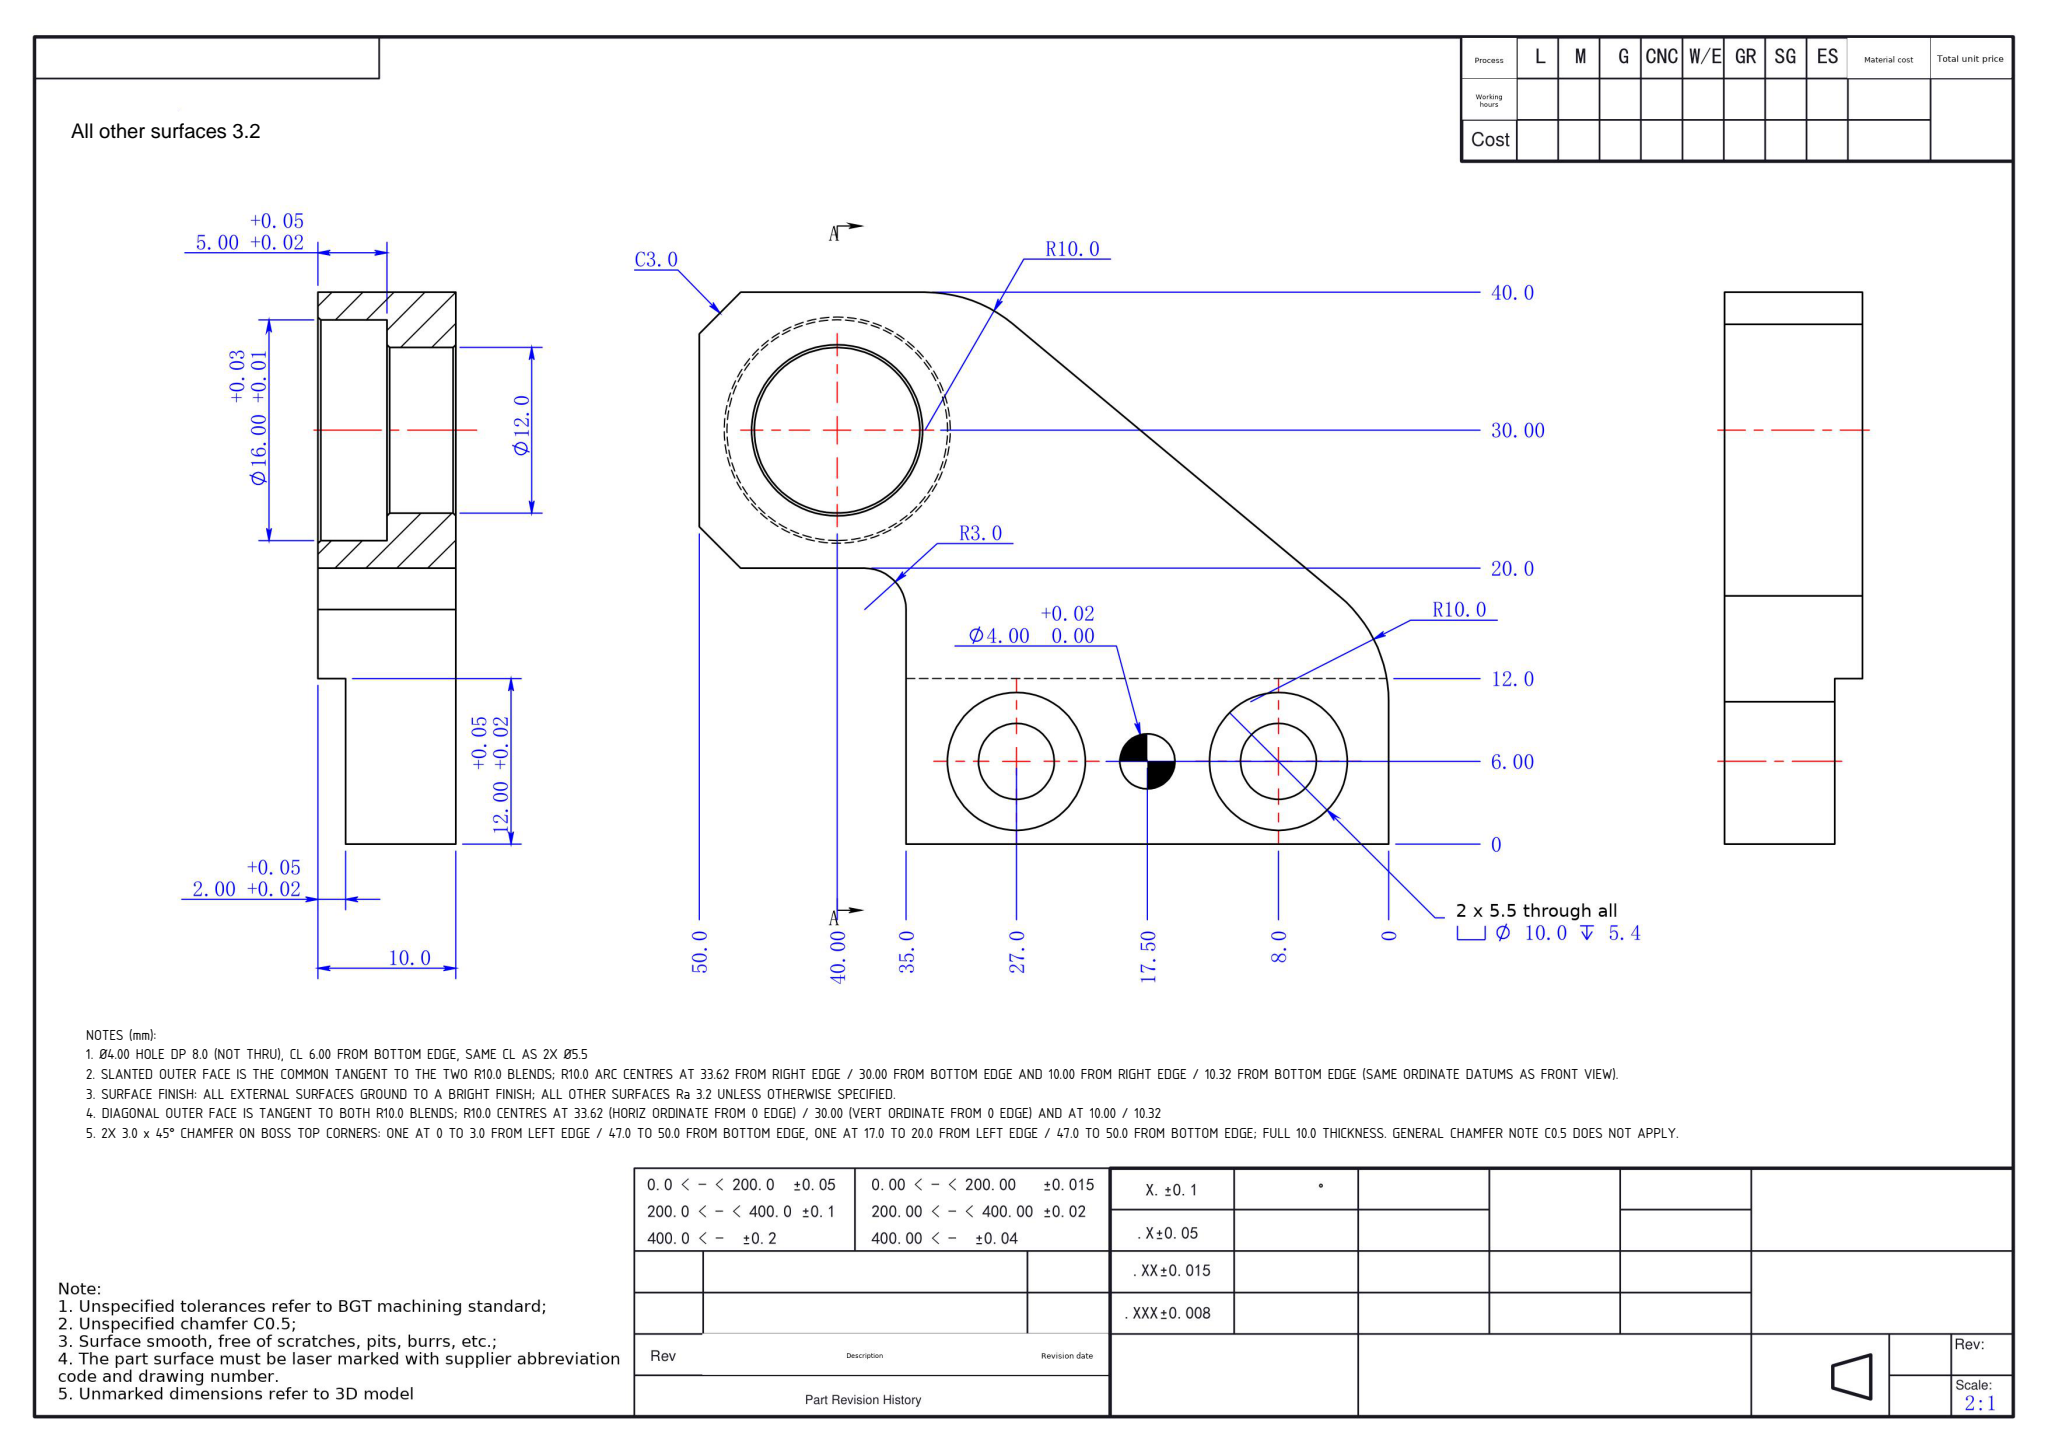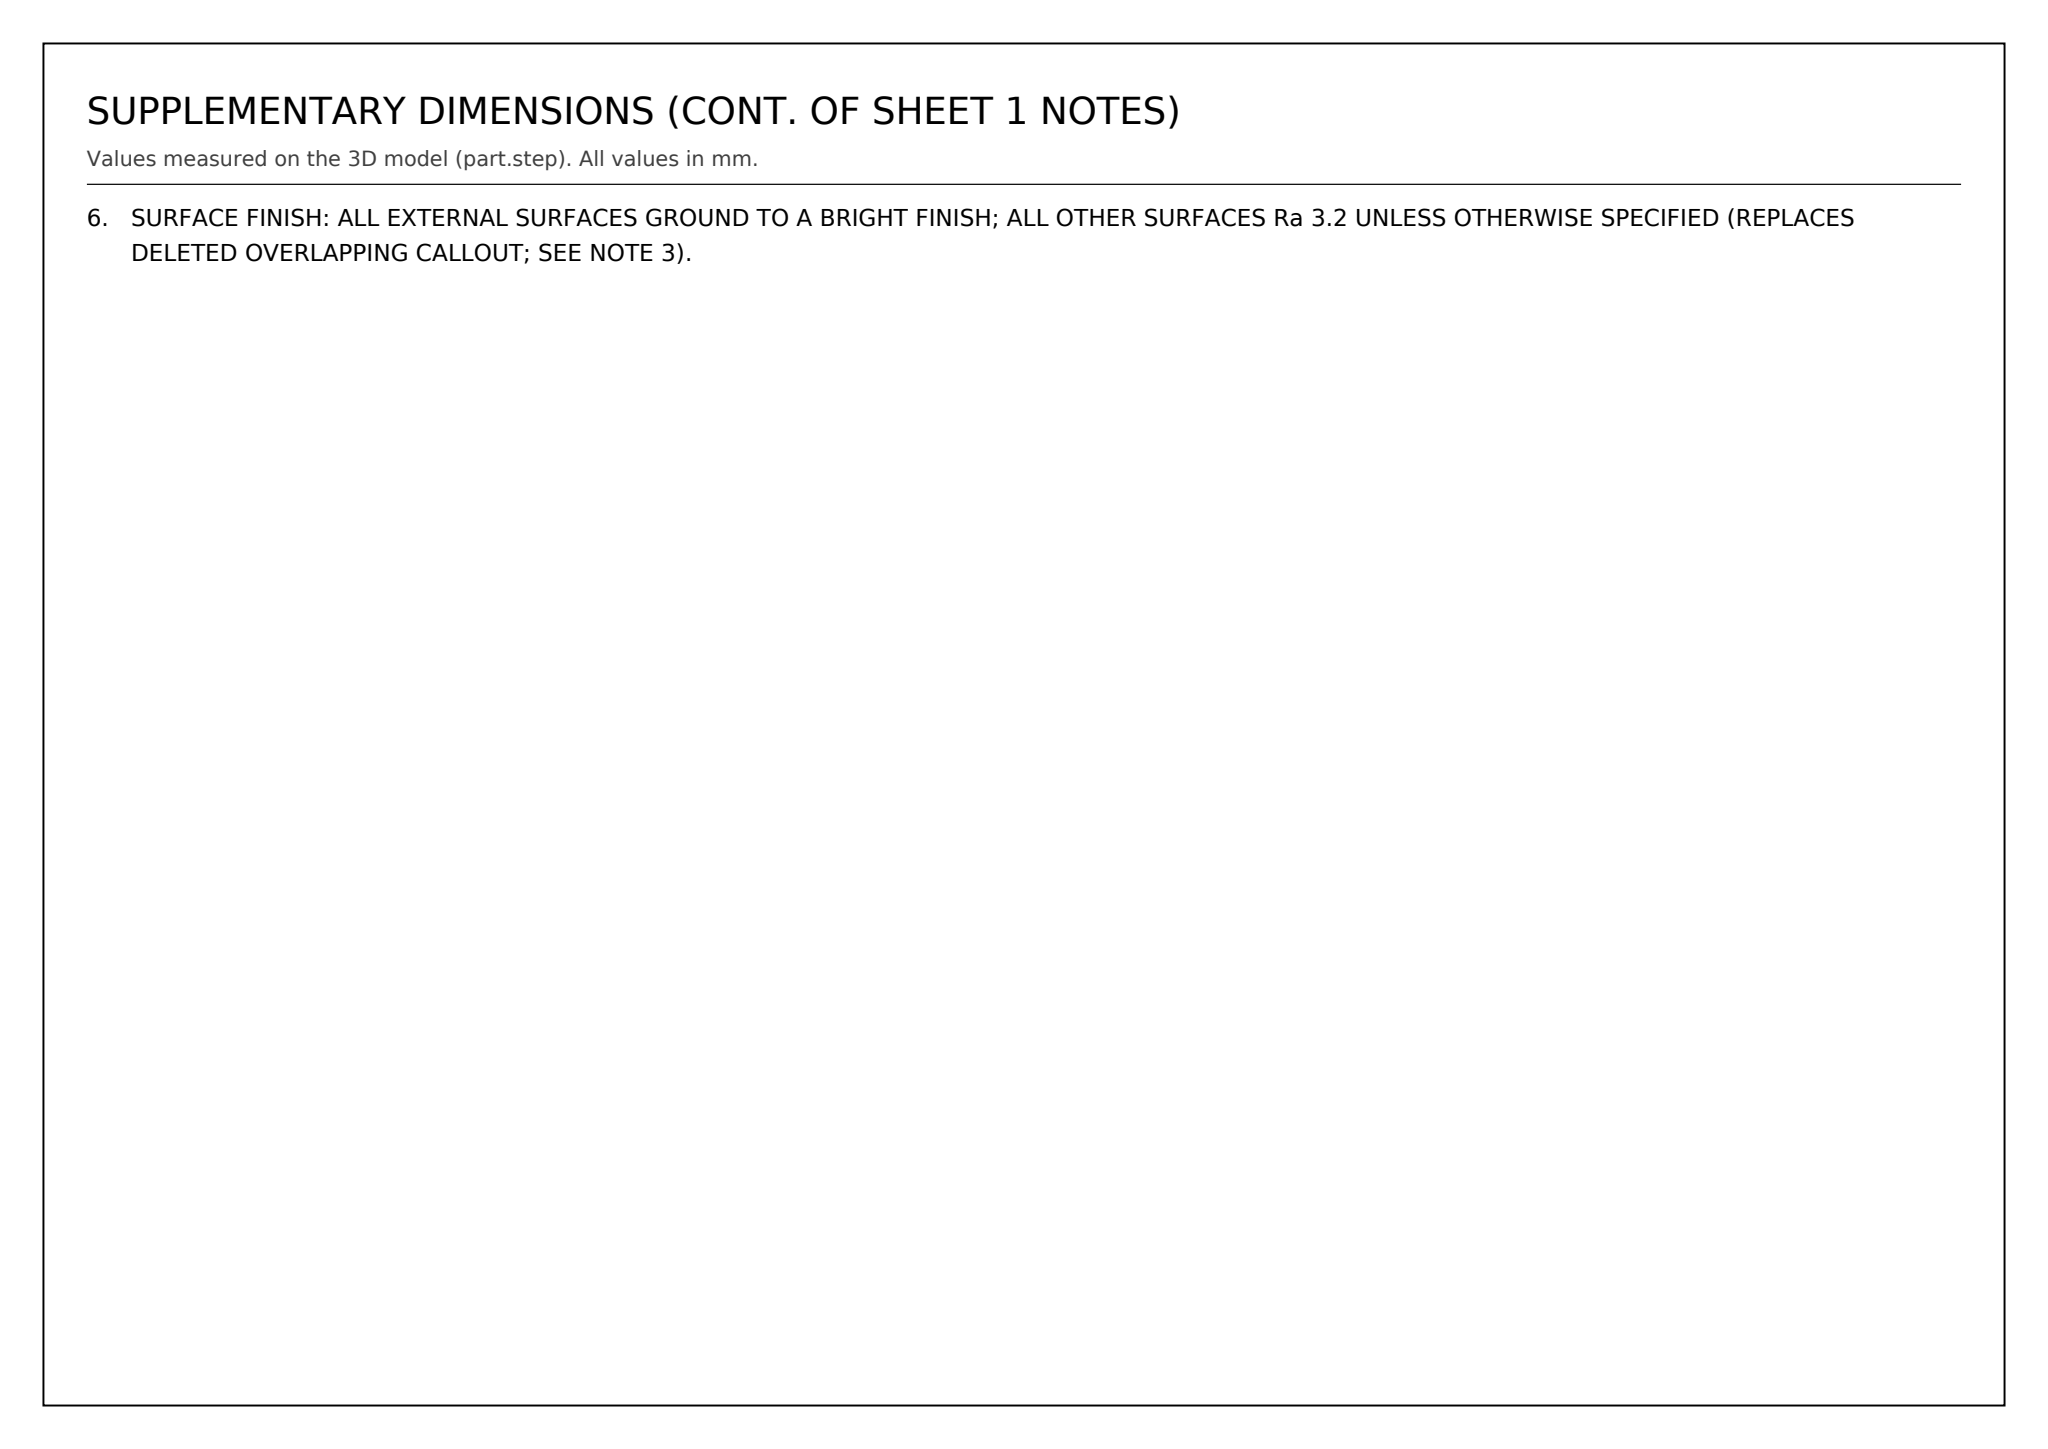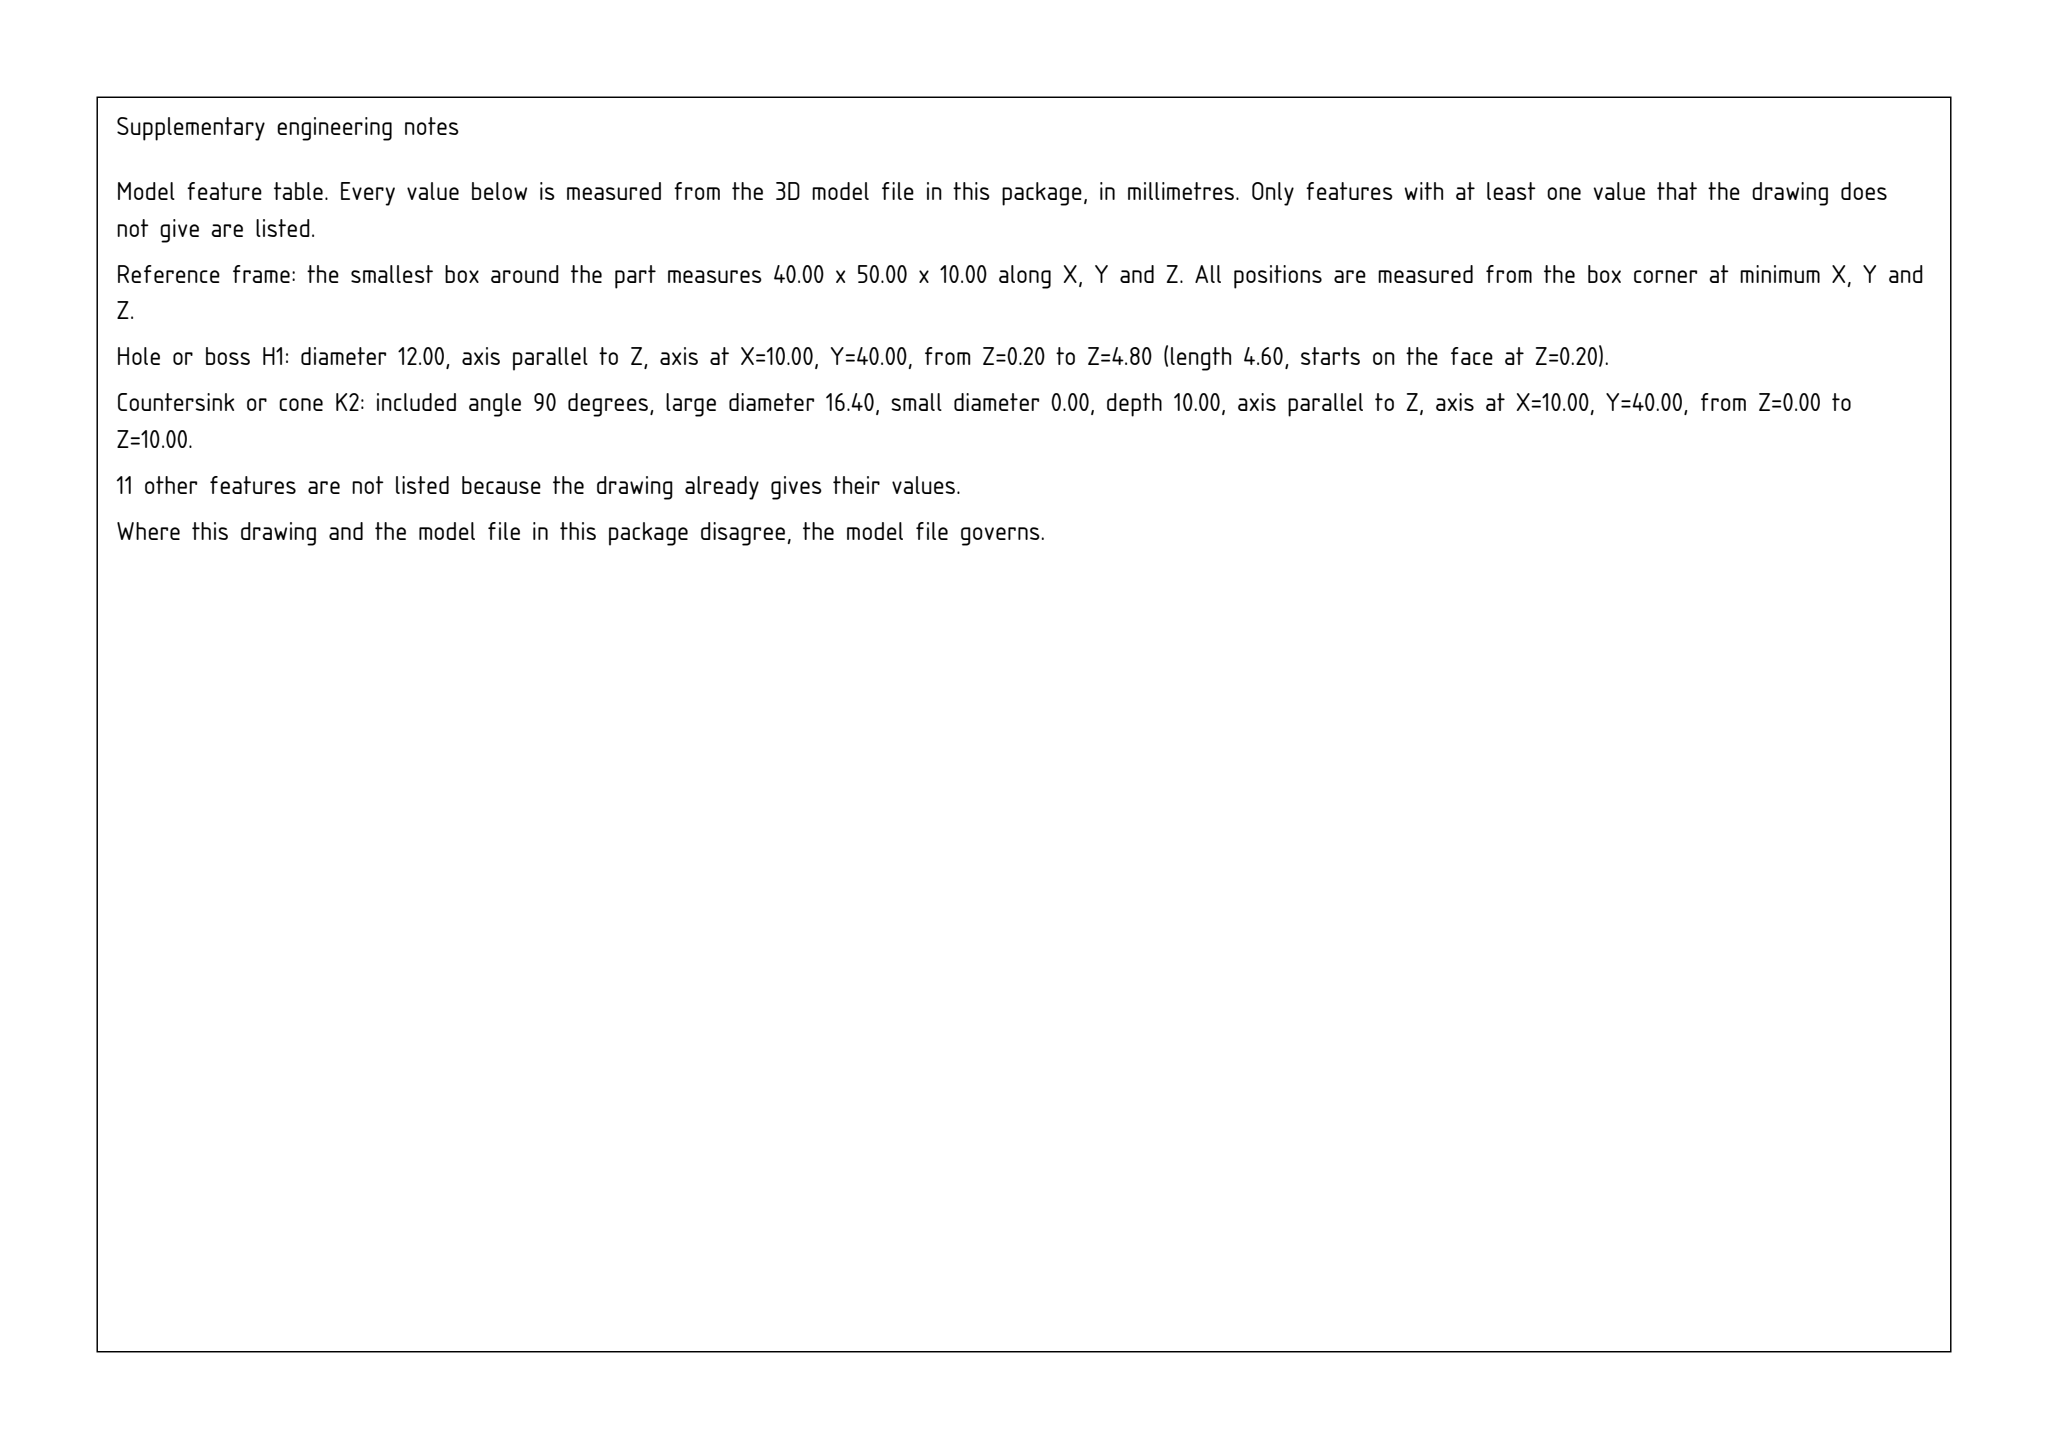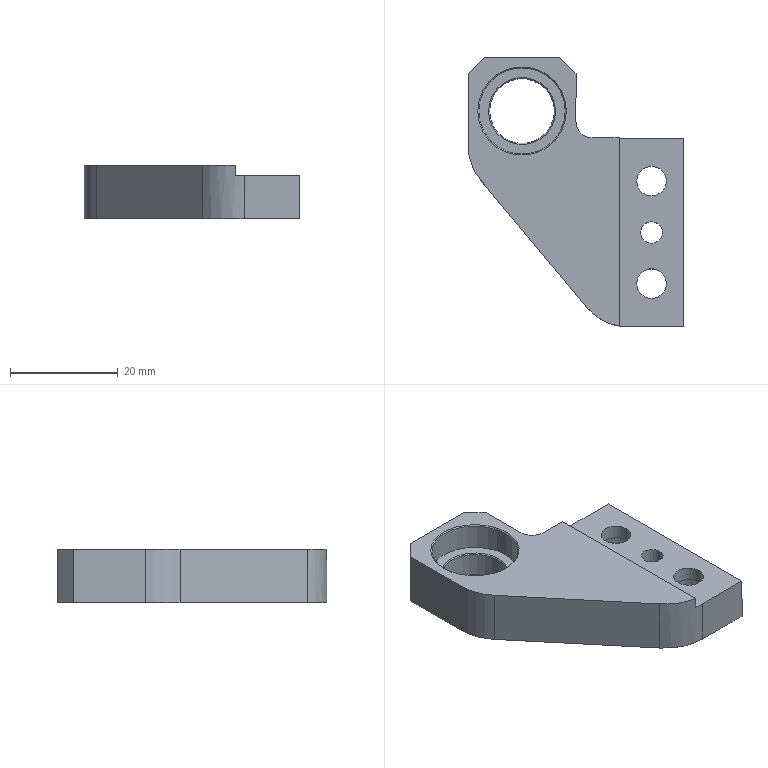Part | SolidWorks | mm | 1 solid | 39 faces | box 40 x 50 x 10 mm | volume 9649 mm3 | cylinder 17 | plane 16 | cone 6 | commonest cylinder face diameters 10 x4 5.5 x4 4 x2 12 x2 16 x2 20 x2 6 x1
Drawing notes:
Ø4.00 HOLE DP 8.0 (NOT THRU), CL 6.00 FROM BOTTOM EDGE, SAME CL AS 2X Ø5.5 | from the solid: cyl dia 4.0 axis z at [34.0,17.5] length 8.0, z-plane at 8.0; bbox x=40 -> 40-34=6.00 from bottom edge; Ø5.5 holes also at x=34
SLANTED OUTER FACE IS THE COMMON TANGENT TO THE TWO R10.0 BLENDS; R10.0 ARC CENTRES AT 33.62 FROM RIGHT EDGE / 30.00 FROM BOTTOM EDGE AND 10.00 FROM RIGHT EDGE / 10.32 FROM BOTTOM EDGE (SAME ORDINATE DATUMS AS FRONT VIEW). | from the solid: cylinders: [20.0,"z",[10.0,33.62],10.0] and [20.0,"z",[29.68,10.0],10.0] (R10 blends, full part thickness 10.0); bbox 40.0 x 50.0 x 10.0
SURFACE FINISH: ALL EXTERNAL SURFACES GROUND TO A BRIGHT FINISH; ALL OTHER SURFACES Ra 3.2 UNLESS OTHERWISE SPECIFIED. | from the solid: no geometry value involved - text restored from the redacted garbled/overlapping surface-finish callout
DIAGONAL OUTER FACE IS TANGENT TO BOTH R10.0 BLENDS; R10.0 CENTRES AT 33.62 (HORIZ ORDINATE FROM 0 EDGE) / 30.00 (VERT ORDINATE FROM 0 EDGE) AND AT 10.00 / 10.32 | from the solid: cylinders dia 20.0 (=R10.0) axis z at [x10.0, y33.62] and [x29.68, y10.0], full 10.0 thickness; bbox 40.0 x 50.0 x 10.0, positions from min corner
2X 3.0 x 45° CHAMFER ON BOSS TOP CORNERS: ONE AT 0 TO 3.0 FROM LEFT EDGE / 47.0 TO 50.0 FROM BOTTOM EDGE, ONE AT 17.0 TO 20.0 FROM LEFT EDGE / 47.0 TO 50.0 FROM BOTTOM EDGE; FULL 10.0 THICKNESS. GENERAL CHAMFER NOTE C0.5 DOES NOT APPLY. | from the solid: inclined_planes: two 45.0/45.0/90.0 faces, bbox_from [0.0,47.0,0.0] and [17.0,47.0,0.0], each size [3.0,3.0,10.0]
SURFACE FINISH: ALL EXTERNAL SURFACES GROUND TO A BRIGHT FINISH; ALL OTHER SURFACES Ra 3.2 UNLESS OTHERWISE SPECIFIED (REPLACES DELETED OVERLAPPING CALLOUT; SEE NOTE 3). | from the solid: no STEP geometry value involved; restores text lost by redaction of the garbled overlapping callout
build123d program:
from build123d import *

# Parameters (mm, degrees)
SKETCH1_W                                       = 40
SKETCH1_H                                       = 50
BOSS_EXTRUDE1_DEPTH                             = 10
SKETCH2_R                                       = 8
CUT_EXTRUDE1_DEPTH                              = 5
SKETCH3_R                                       = 6
CUT_EXTRUDE2_DEPTH                              = 65.226
SKETCH4_W                                       = 20
SKETCH4_H                                       = 15
CUT_EXTRUDE3_DEPTH                              = 65.807
CHAMFER1_SIZE                                   = 3
SKETCH5_W                                       = 12
SKETCH5_H                                       = 35
BOSS_EXTRUDE2_DEPTH                             = 32
M5_HEX_SOCKET_HEAD_CAP_SCREW_CBORE1_D           = 5.5
M5_HEX_SOCKET_HEAD_CAP_SCREW_CBORE1_CBORE_D     = 10
M5_HEX_SOCKET_HEAD_CAP_SCREW_CBORE1_CBORE_DEPTH = 5.4
CHAMFER2_SIZE                                   = 30
CHAMFER2_SIZE2                                  = 25
SKETCH8_W                                       = 12
SKETCH8_H                                       = 32
CUT_EXTRUDE4_DEPTH                              = 77.577
SKETCH9_W                                       = 12
SKETCH9_H                                       = 2
CUT_EXTRUDE5_DEPTH                              = 65.807
FILLET1_R                                       = 3
FILLET2_R                                       = 10
CHAMFER3_SIZE                                   = 0.2
SIZE_MM_DOWEL_PIN_HOLE1_D                       = 4


with BuildPart() as part:
    # Sketch1 → Boss-Extrude1 (new body)
    with BuildSketch(Plane.XY):
        with Locations((20, 25)):
            Rectangle(SKETCH1_W, SKETCH1_H)
    extrude(amount=BOSS_EXTRUDE1_DEPTH)

    # Sketch2 → Cut-Extrude1 (cut)
    with BuildSketch(Plane.XY.offset(10)):
        with Locations((10, 40)):
            Circle(SKETCH2_R)
    extrude(amount=-CUT_EXTRUDE1_DEPTH, mode=Mode.SUBTRACT)

    # Sketch3 → Cut-Extrude2 (cut, through all)
    with BuildSketch(Plane.XY.offset(5)):
        with Locations((10, 40)):
            Circle(SKETCH3_R)
    extrude(amount=-CUT_EXTRUDE2_DEPTH, mode=Mode.SUBTRACT)

    # Sketch4 → Cut-Extrude3 (cut, through all)
    with BuildSketch(Plane(origin=(0, 0, 0), x_dir=(-1, 0, 0), z_dir=(0, 0, -1))):
        with Locations((-30, 42.5)):
            Rectangle(SKETCH4_W, SKETCH4_H)
    extrude(amount=-CUT_EXTRUDE3_DEPTH, mode=Mode.SUBTRACT)

    # Chamfer1
    chamfer1_edges = [part.edges().sort_by_distance(p)[0] for p in [
        (20, 50, 5),
        (0, 50, 5),
    ]]
    chamfer(chamfer1_edges, length=CHAMFER1_SIZE)

    # Sketch5 → Boss-Extrude2 (add)
    with BuildSketch(Plane.XY.offset(10)):
        with Locations((34, 17.5)):
            Rectangle(SKETCH5_W, SKETCH5_H)
    extrude(amount=BOSS_EXTRUDE2_DEPTH)

    # M5 Hex Socket Head Cap Screw CBORE1 (through all)
    with Locations(Plane(origin=(0, 0, 0), x_dir=(-1, 0, 0), z_dir=(0, 0, -1))):
        with Locations((-34, 27), (-34, 8)):
            CounterBoreHole(M5_HEX_SOCKET_HEAD_CAP_SCREW_CBORE1_D / 2, M5_HEX_SOCKET_HEAD_CAP_SCREW_CBORE1_CBORE_D / 2, M5_HEX_SOCKET_HEAD_CAP_SCREW_CBORE1_CBORE_DEPTH)

    # Chamfer2
    chamfer2_edges = [part.edges().sort_by_distance(p)[0] for p in [
        (0, 0, 5),
    ]]
    chamfer2_side = [part.faces().sort_by_distance(p)[0] for p in [
        (0, 23.5, 5),
    ]]
    chamfer(chamfer2_edges, length=CHAMFER2_SIZE, length2=CHAMFER2_SIZE2, reference=chamfer2_side[0])

    # Sketch8 → Cut-Extrude4 (cut, through all)
    with BuildSketch(Plane(origin=(0, 0, 0), x_dir=(-1, 0, 0), z_dir=(0, -1, 0))):
        with Locations((-34, -26)):
            Rectangle(SKETCH8_W, SKETCH8_H)
    extrude(amount=-CUT_EXTRUDE4_DEPTH, mode=Mode.SUBTRACT)

    # Sketch9 → Cut-Extrude5 (cut, through all)
    with BuildSketch(Plane.XZ):
        with Locations((34, 9)):
            Rectangle(SKETCH9_W, SKETCH9_H)
    extrude(amount=-CUT_EXTRUDE5_DEPTH, mode=Mode.SUBTRACT)

    # Fillet1
    fillet1_edges = [part.edges().sort_by_distance(p)[0] for p in [
        (20, 35, 5),
    ]]
    fillet(fillet1_edges, radius=FILLET1_R)

    # Fillet2
    fillet2_edges = [part.edges().sort_by_distance(p)[0] for p in [
        (25, 0, 5),
        (0, 30, 5),
    ]]
    fillet(fillet2_edges, radius=FILLET2_R)

    # Chamfer3
    chamfer3_edges = [part.edges().sort_by_distance(p)[0] for p in [
        (2, 40, 10),
        (4, 40, 0),
        (4, 40, 5),
    ]]
    chamfer(chamfer3_edges, length=CHAMFER3_SIZE)

    # Size mm Dowel Pin Hole1 (through all)
    with Locations(Plane(origin=(0, 0, 0), x_dir=(-1, 0, 0), z_dir=(0, 0, -1))):
        with Locations((-34, 17.5)):
            Hole(SIZE_MM_DOWEL_PIN_HOLE1_D / 2)


solid = part.part